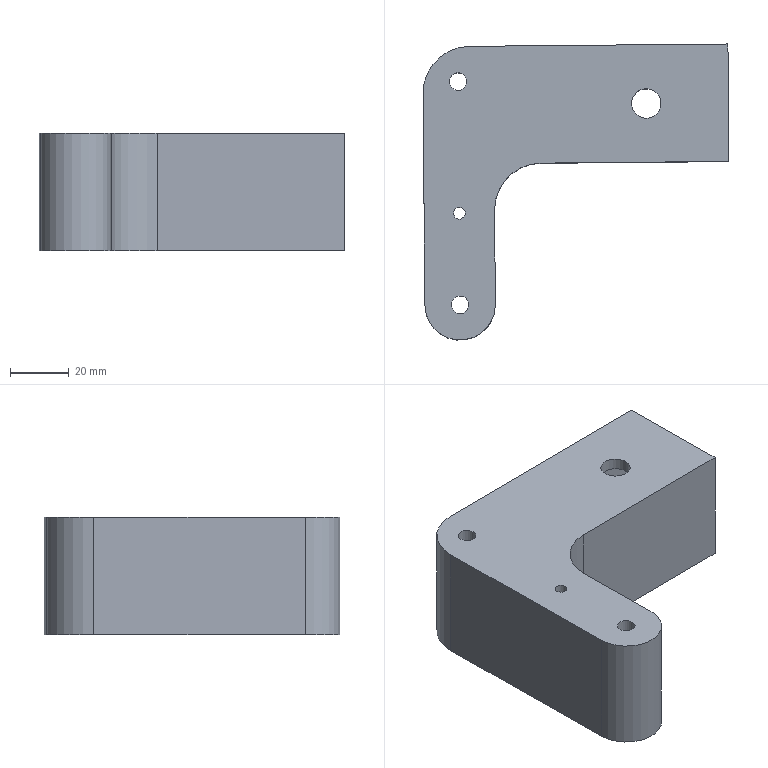Component | NX | 5 | 1 solid | 20 faces | volume 168983 mm3 | plane 12 | cylinder 8 | commonest cylinder face diameters 10 x2 32 x2 6 x2 24 x1 4 x1